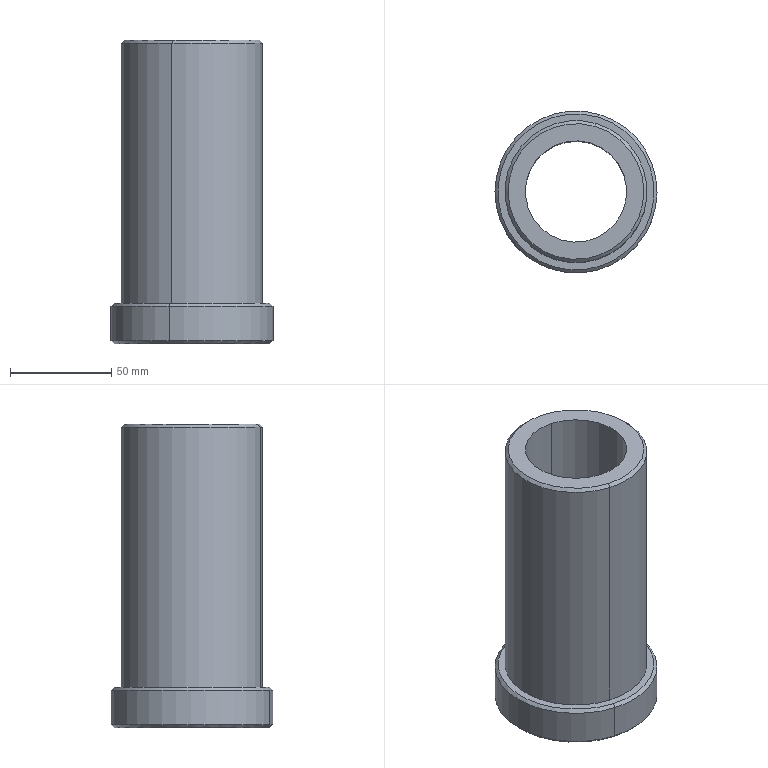Component | SolidWorks | GuideBushing-2 | 1 solid | 15 faces | box 80 x 80 x 150 mm | volume 305503 mm3 | cone 6 | cylinder 6 | plane 3 | commonest cylinder face diameters 50 x2 70 x2 80 x2
build123d program:
from build123d import *

# Parameters (mm, degrees)
CUT_EXTRUDE1_DEPTH      = 161.312
CUT_EXTRUDE1_DEPTH_BACK = 161.312
SKETCH2_R               = 25
CHAMFER1_SIZE           = 1.5


with BuildPart() as part:
    # Sketch1 → Revolve1 (revolve)
    with BuildSketch(Plane.XY, mode=Mode.PRIVATE) as revolve1_sk:
        Polygon((0, 0), (0, 150), (40, 150), (40, 130), (35, 130), (35, 0), align=None)
    revolve(revolve1_sk.sketch.rotate(Axis((0, 0, 0), (0, 1, 0)), 90), axis=Axis((0, 0, 0), (0, 1, 0)))

    # Sketch2 → Cut-Extrude1 (cut, two sides: drawn at the far end of the back side and taken through both)
    with BuildSketch(Plane(origin=(0, 150, 0), x_dir=(1, 0, 0), z_dir=(0, 1, 0)).offset(-CUT_EXTRUDE1_DEPTH_BACK)):
        with Locations(Location((0, 0, 0), (0, 0, 270))):
            Circle(SKETCH2_R)
    extrude(amount=CUT_EXTRUDE1_DEPTH + CUT_EXTRUDE1_DEPTH_BACK, mode=Mode.SUBTRACT)

    # Chamfer1
    chamfer1_edges = [part.edges().sort_by_distance(p)[0] for p in [
        (0, 0, 35),
        (0, 130, 40),
        (0, 150, 40),
    ]]
    chamfer(chamfer1_edges, length=CHAMFER1_SIZE)


solid = part.part

# Placed as in the assembly
solid = solid.moved(Location((-195, 195, -191), (-90, 0, 0)))
STEP:
#1=CARTESIAN_POINT('',(-7.248,9.131,-13.425));
#2=VERTEX_POINT('',#1);
#3=CARTESIAN_POINT('',(-8.106,6.223,-13.425));
#4=VERTEX_POINT('',#3);
#5=CARTESIAN_POINT('',(-7.677,7.677,-13.425));
#6=DIRECTION('',(-0.,0.,-1.));
#7=DIRECTION('',(0.283,0.9591,0.));
#8=AXIS2_PLACEMENT_3D('',#5,#6,#7);
#9=CIRCLE('',#8,1.516);
#10=EDGE_CURVE('',#2,#4,#9,.T.);
#11=ORIENTED_EDGE('',*,*,#10,.F.);
#12=CARTESIAN_POINT('',(-7.232,9.188,-13.366));
#13=VERTEX_POINT('',#12);
#14=CARTESIAN_POINT('',(-7.232,9.188,-13.366));
#15=DIRECTION('',(0.2001,0.6782,0.7071));
#16=VECTOR('',#15,39.37);
#17=LINE('',#14,#16);
#18=EDGE_CURVE('',#2,#13,#17,.T.);
#19=ORIENTED_EDGE('',*,*,#18,.T.);
#20=CARTESIAN_POINT('',(-8.123,6.167,-13.366));
#21=VERTEX_POINT('',#20);
#22=CARTESIAN_POINT('',(-7.677,7.677,-13.366));
#23=DIRECTION('',(0.,-0.,1.));
#24=DIRECTION('',(0.283,0.9591,0.));
#25=AXIS2_PLACEMENT_3D('',#22,#23,#24);
#26=CIRCLE('',#25,1.575);
#27=EDGE_CURVE('',#21,#13,#26,.T.);
#28=ORIENTED_EDGE('',*,*,#27,.F.);
#29=CARTESIAN_POINT('',(-8.123,6.167,-13.366));
#30=DIRECTION('',(-0.2001,-0.6782,0.7071));
#31=VECTOR('',#30,39.37);
#32=LINE('',#29,#31);
#33=EDGE_CURVE('',#4,#21,#32,.T.);
#34=ORIENTED_EDGE('',*,*,#33,.F.);
#35=EDGE_LOOP('',(#11,#19,#28,#34));
#36=FACE_OUTER_BOUND('',#35,.T.);
#37=CARTESIAN_POINT('',(-7.677,7.677,-13.366));
#38=DIRECTION('',(0.,-0.,1.));
#39=DIRECTION('',(-0.283,-0.9591,0.));
#40=AXIS2_PLACEMENT_3D('',#37,#38,#39);
#41=CONICAL_SURFACE('',#40,1.575,0.7854);
#42=ADVANCED_FACE('',(#36),#41,.T.);
#43=CARTESIAN_POINT('',(-8.106,6.223,-12.638));
#44=VERTEX_POINT('',#43);
#45=CARTESIAN_POINT('',(-7.248,9.131,-12.638));
#46=VERTEX_POINT('',#45);
#47=CARTESIAN_POINT('',(-7.677,7.677,-12.638));
#48=DIRECTION('',(0.,-0.,1.));
#49=DIRECTION('',(-0.283,-0.9591,0.));
#50=AXIS2_PLACEMENT_3D('',#47,#48,#49);
#51=CIRCLE('',#50,1.516);
#52=EDGE_CURVE('',#44,#46,#51,.T.);
#53=ORIENTED_EDGE('',*,*,#52,.F.);
#54=CARTESIAN_POINT('',(-8.123,6.167,-12.697));
#55=VERTEX_POINT('',#54);
#56=CARTESIAN_POINT('',(-8.106,6.223,-12.638));
#57=DIRECTION('',(-0.2001,-0.6782,-0.7071));
#58=VECTOR('',#57,39.37);
#59=LINE('',#56,#58);
#60=EDGE_CURVE('',#44,#55,#59,.T.);
#61=ORIENTED_EDGE('',*,*,#60,.T.);
#62=CARTESIAN_POINT('',(-7.232,9.188,-12.697));
#63=VERTEX_POINT('',#62);
#64=CARTESIAN_POINT('',(-7.677,7.677,-12.697));
#65=DIRECTION('',(-0.,0.,-1.));
#66=DIRECTION('',(-0.283,-0.9591,0.));
#67=AXIS2_PLACEMENT_3D('',#64,#65,#66);
#68=CIRCLE('',#67,1.575);
#69=EDGE_CURVE('',#63,#55,#68,.T.);
#70=ORIENTED_EDGE('',*,*,#69,.F.);
#71=CARTESIAN_POINT('',(-7.248,9.131,-12.638));
#72=DIRECTION('',(0.2001,0.6782,-0.7071));
#73=VECTOR('',#72,39.37);
#74=LINE('',#71,#73);
#75=EDGE_CURVE('',#46,#63,#74,.T.);
#76=ORIENTED_EDGE('',*,*,#75,.F.);
#77=EDGE_LOOP('',(#53,#61,#70,#76));
#78=FACE_OUTER_BOUND('',#77,.T.);
#79=CARTESIAN_POINT('',(-7.677,7.677,-12.638));
#80=DIRECTION('',(-0.,0.,-1.));
#81=DIRECTION('',(0.283,0.9591,0.));
#82=AXIS2_PLACEMENT_3D('',#79,#80,#81);
#83=CONICAL_SURFACE('',#82,1.516,0.7854);
#84=ADVANCED_FACE('',(#78),#83,.T.);
#85=CARTESIAN_POINT('',(-8.05,6.412,-7.52));
#86=VERTEX_POINT('',#85);
#87=CARTESIAN_POINT('',(-7.304,8.942,-7.52));
#88=VERTEX_POINT('',#87);
#89=CARTESIAN_POINT('',(-7.677,7.677,-7.52));
#90=DIRECTION('',(0.,-0.,1.));
#91=DIRECTION('',(-0.283,-0.9591,0.));
#92=AXIS2_PLACEMENT_3D('',#89,#90,#91);
#93=CIRCLE('',#92,1.319);
#94=EDGE_CURVE('',#86,#88,#93,.T.);
#95=ORIENTED_EDGE('',*,*,#94,.F.);
#96=CARTESIAN_POINT('',(-8.067,6.356,-7.579));
#97=VERTEX_POINT('',#96);
#98=CARTESIAN_POINT('',(-8.05,6.412,-7.52));
#99=DIRECTION('',(-0.2001,-0.6782,-0.7071));
#100=VECTOR('',#99,39.37);
#101=LINE('',#98,#100);
#102=EDGE_CURVE('',#86,#97,#101,.T.);
#103=ORIENTED_EDGE('',*,*,#102,.T.);
#104=CARTESIAN_POINT('',(-7.287,8.999,-7.579));
#105=VERTEX_POINT('',#104);
#106=CARTESIAN_POINT('',(-7.677,7.677,-7.579));
#107=DIRECTION('',(-0.,0.,-1.));
#108=DIRECTION('',(-0.283,-0.9591,0.));
#109=AXIS2_PLACEMENT_3D('',#106,#107,#108);
#110=CIRCLE('',#109,1.378);
#111=EDGE_CURVE('',#105,#97,#110,.T.);
#112=ORIENTED_EDGE('',*,*,#111,.F.);
#113=CARTESIAN_POINT('',(-7.304,8.942,-7.52));
#114=DIRECTION('',(0.2001,0.6782,-0.7071));
#115=VECTOR('',#114,39.37);
#116=LINE('',#113,#115);
#117=EDGE_CURVE('',#88,#105,#116,.T.);
#118=ORIENTED_EDGE('',*,*,#117,.F.);
#119=EDGE_LOOP('',(#95,#103,#112,#118));
#120=FACE_OUTER_BOUND('',#119,.T.);
#121=CARTESIAN_POINT('',(-7.677,7.677,-7.52));
#122=DIRECTION('',(-0.,0.,-1.));
#123=DIRECTION('',(0.283,0.9591,0.));
#124=AXIS2_PLACEMENT_3D('',#121,#122,#123);
#125=CONICAL_SURFACE('',#124,1.319,0.7854);
#126=ADVANCED_FACE('',(#120),#125,.T.);
#127=CARTESIAN_POINT('',(-7.956,6.733,-7.52));
#128=VERTEX_POINT('',#127);
#129=CARTESIAN_POINT('',(-7.399,8.621,-7.52));
#130=VERTEX_POINT('',#129);
#131=CARTESIAN_POINT('',(-7.677,7.677,-7.52));
#132=DIRECTION('',(-0.,0.,-1.));
#133=DIRECTION('',(0.283,0.9591,0.));
#134=AXIS2_PLACEMENT_3D('',#131,#132,#133);
#135=CIRCLE('',#134,0.9843);
#136=EDGE_CURVE('',#128,#130,#135,.T.);
#137=ORIENTED_EDGE('',*,*,#136,.F.);
#138=CARTESIAN_POINT('',(-7.956,6.733,-13.425));
#139=VERTEX_POINT('',#138);
#140=CARTESIAN_POINT('',(-7.956,6.733,-7.52));
#141=DIRECTION('',(-0.,0.,-1.));
#142=VECTOR('',#141,39.37);
#143=LINE('',#140,#142);
#144=EDGE_CURVE('',#128,#139,#143,.T.);
#145=ORIENTED_EDGE('',*,*,#144,.T.);
#146=CARTESIAN_POINT('',(-7.399,8.621,-13.425));
#147=VERTEX_POINT('',#146);
#148=CARTESIAN_POINT('',(-7.677,7.677,-13.425));
#149=DIRECTION('',(-0.,0.,-1.));
#150=DIRECTION('',(0.283,0.9591,0.));
#151=AXIS2_PLACEMENT_3D('',#148,#149,#150);
#152=CIRCLE('',#151,0.9843);
#153=EDGE_CURVE('',#139,#147,#152,.T.);
#154=ORIENTED_EDGE('',*,*,#153,.T.);
#155=CARTESIAN_POINT('',(-7.399,8.621,-7.52));
#156=DIRECTION('',(-0.,0.,-1.));
#157=VECTOR('',#156,39.37);
#158=LINE('',#155,#157);
#159=EDGE_CURVE('',#130,#147,#158,.T.);
#160=ORIENTED_EDGE('',*,*,#159,.F.);
#161=EDGE_LOOP('',(#137,#145,#154,#160));
#162=FACE_OUTER_BOUND('',#161,.T.);
#163=CARTESIAN_POINT('',(-7.677,7.677,-7.52));
#164=DIRECTION('',(-0.,0.,-1.));
#165=DIRECTION('',(0.283,0.9591,0.));
#166=AXIS2_PLACEMENT_3D('',#163,#164,#165);
#167=CYLINDRICAL_SURFACE('',#166,0.9843);
#168=ADVANCED_FACE('',(#162),#167,.F.);
#169=CARTESIAN_POINT('',(-8.067,6.356,-12.638));
#170=VERTEX_POINT('',#169);
#171=CARTESIAN_POINT('',(-7.287,8.999,-12.638));
#172=VERTEX_POINT('',#171);
#173=CARTESIAN_POINT('',(-7.677,7.677,-12.638));
#174=DIRECTION('',(0.,-0.,1.));
#175=DIRECTION('',(-0.283,-0.9591,0.));
#176=AXIS2_PLACEMENT_3D('',#173,#174,#175);
#177=CIRCLE('',#176,1.378);
#178=EDGE_CURVE('',#170,#172,#177,.T.);
#179=ORIENTED_EDGE('',*,*,#178,.T.);
#180=CARTESIAN_POINT('',(-7.287,8.999,-7.52));
#181=DIRECTION('',(0.,-0.,1.));
#182=VECTOR('',#181,39.37);
#183=LINE('',#180,#182);
#184=EDGE_CURVE('',#172,#105,#183,.T.);
#185=ORIENTED_EDGE('',*,*,#184,.T.);
#186=ORIENTED_EDGE('',*,*,#111,.T.);
#187=CARTESIAN_POINT('',(-8.067,6.356,-7.52));
#188=DIRECTION('',(0.,-0.,1.));
#189=VECTOR('',#188,39.37);
#190=LINE('',#187,#189);
#191=EDGE_CURVE('',#170,#97,#190,.T.);
#192=ORIENTED_EDGE('',*,*,#191,.F.);
#193=EDGE_LOOP('',(#179,#185,#186,#192));
#194=FACE_OUTER_BOUND('',#193,.T.);
#195=CARTESIAN_POINT('',(-7.677,7.677,-7.52));
#196=DIRECTION('',(0.,-0.,1.));
#197=DIRECTION('',(-0.283,-0.9591,0.));
#198=AXIS2_PLACEMENT_3D('',#195,#196,#197);
#199=CYLINDRICAL_SURFACE('',#198,1.378);
#200=ADVANCED_FACE('',(#194),#199,.T.);
#201=ORIENTED_EDGE('',*,*,#27,.T.);
#202=CARTESIAN_POINT('',(-7.232,9.188,-7.52));
#203=DIRECTION('',(0.,-0.,1.));
#204=VECTOR('',#203,39.37);
#205=LINE('',#202,#204);
#206=EDGE_CURVE('',#13,#63,#205,.T.);
#207=ORIENTED_EDGE('',*,*,#206,.T.);
#208=ORIENTED_EDGE('',*,*,#69,.T.);
#209=CARTESIAN_POINT('',(-8.123,6.167,-7.52));
#210=DIRECTION('',(0.,-0.,1.));
#211=VECTOR('',#210,39.37);
#212=LINE('',#209,#211);
#213=EDGE_CURVE('',#21,#55,#212,.T.);
#214=ORIENTED_EDGE('',*,*,#213,.F.);
#215=EDGE_LOOP('',(#201,#207,#208,#214));
#216=FACE_OUTER_BOUND('',#215,.T.);
#217=CARTESIAN_POINT('',(-7.677,7.677,-7.52));
#218=DIRECTION('',(0.,-0.,1.));
#219=DIRECTION('',(-0.283,-0.9591,0.));
#220=AXIS2_PLACEMENT_3D('',#217,#218,#219);
#221=CYLINDRICAL_SURFACE('',#220,1.575);
#222=ADVANCED_FACE('',(#216),#221,.T.);
#223=CARTESIAN_POINT('',(-7.677,7.677,-7.52));
#224=DIRECTION('',(0.,-0.,1.));
#225=DIRECTION('',(-0.283,-0.9591,0.));
#226=AXIS2_PLACEMENT_3D('',#223,#224,#225);
#227=CIRCLE('',#226,1.319);
#228=EDGE_CURVE('',#88,#86,#227,.T.);
#229=ORIENTED_EDGE('',*,*,#228,.T.);
#230=ORIENTED_EDGE('',*,*,#94,.T.);
#231=EDGE_LOOP('',(#229,#230));
#232=FACE_OUTER_BOUND('',#231,.T.);
#233=CARTESIAN_POINT('',(-7.677,7.677,-7.52));
#234=DIRECTION('',(-0.,0.,-1.));
#235=DIRECTION('',(0.283,0.9591,0.));
#236=AXIS2_PLACEMENT_3D('',#233,#234,#235);
#237=CIRCLE('',#236,0.9843);
#238=EDGE_CURVE('',#130,#128,#237,.T.);
#239=ORIENTED_EDGE('',*,*,#238,.T.);
#240=ORIENTED_EDGE('',*,*,#136,.T.);
#241=EDGE_LOOP('',(#239,#240));
#242=FACE_BOUND('',#241,.T.);
#243=CARTESIAN_POINT('',(-6.356,7.287,-7.52));
#244=DIRECTION('',(0.,-0.,1.));
#245=DIRECTION('',(-0.283,-0.9591,0.));
#246=AXIS2_PLACEMENT_3D('',#243,#244,#245);
#247=PLANE('',#246);
#248=ADVANCED_FACE('',(#232,#242),#247,.T.);
#249=CARTESIAN_POINT('',(-7.677,7.677,-13.425));
#250=DIRECTION('',(-0.,0.,-1.));
#251=DIRECTION('',(0.283,0.9591,0.));
#252=AXIS2_PLACEMENT_3D('',#249,#250,#251);
#253=CIRCLE('',#252,1.516);
#254=EDGE_CURVE('',#4,#2,#253,.T.);
#255=ORIENTED_EDGE('',*,*,#254,.T.);
#256=ORIENTED_EDGE('',*,*,#10,.T.);
#257=EDGE_LOOP('',(#255,#256));
#258=FACE_OUTER_BOUND('',#257,.T.);
#259=CARTESIAN_POINT('',(-7.677,7.677,-13.425));
#260=DIRECTION('',(-0.,0.,-1.));
#261=DIRECTION('',(0.283,0.9591,0.));
#262=AXIS2_PLACEMENT_3D('',#259,#260,#261);
#263=CIRCLE('',#262,0.9843);
#264=EDGE_CURVE('',#147,#139,#263,.T.);
#265=ORIENTED_EDGE('',*,*,#264,.F.);
#266=ORIENTED_EDGE('',*,*,#153,.F.);
#267=EDGE_LOOP('',(#265,#266));
#268=FACE_BOUND('',#267,.T.);
#269=CARTESIAN_POINT('',(-7.677,7.677,-13.425));
#270=DIRECTION('',(-0.,0.,-1.));
#271=DIRECTION('',(0.283,0.9591,-0.));
#272=AXIS2_PLACEMENT_3D('',#269,#270,#271);
#273=PLANE('',#272);
#274=ADVANCED_FACE('',(#258,#268),#273,.T.);
#275=ORIENTED_EDGE('',*,*,#206,.F.);
#276=CARTESIAN_POINT('',(-7.677,7.677,-13.366));
#277=DIRECTION('',(0.,-0.,1.));
#278=DIRECTION('',(0.283,0.9591,0.));
#279=AXIS2_PLACEMENT_3D('',#276,#277,#278);
#280=CIRCLE('',#279,1.575);
#281=EDGE_CURVE('',#13,#21,#280,.T.);
#282=ORIENTED_EDGE('',*,*,#281,.T.);
#283=ORIENTED_EDGE('',*,*,#213,.T.);
#284=CARTESIAN_POINT('',(-7.677,7.677,-12.697));
#285=DIRECTION('',(-0.,0.,-1.));
#286=DIRECTION('',(-0.283,-0.9591,0.));
#287=AXIS2_PLACEMENT_3D('',#284,#285,#286);
#288=CIRCLE('',#287,1.575);
#289=EDGE_CURVE('',#55,#63,#288,.T.);
#290=ORIENTED_EDGE('',*,*,#289,.T.);
#291=EDGE_LOOP('',(#275,#282,#283,#290));
#292=FACE_OUTER_BOUND('',#291,.T.);
#293=CARTESIAN_POINT('',(-7.677,7.677,-7.52));
#294=DIRECTION('',(0.,-0.,1.));
#295=DIRECTION('',(-0.283,-0.9591,0.));
#296=AXIS2_PLACEMENT_3D('',#293,#294,#295);
#297=CYLINDRICAL_SURFACE('',#296,1.575);
#298=ADVANCED_FACE('',(#292),#297,.T.);
#299=CARTESIAN_POINT('',(-7.677,7.677,-12.638));
#300=DIRECTION('',(0.,-0.,1.));
#301=DIRECTION('',(-0.283,-0.9591,0.));
#302=AXIS2_PLACEMENT_3D('',#299,#300,#301);
#303=CIRCLE('',#302,1.516);
#304=EDGE_CURVE('',#46,#44,#303,.T.);
#305=ORIENTED_EDGE('',*,*,#304,.T.);
#306=ORIENTED_EDGE('',*,*,#52,.T.);
#307=EDGE_LOOP('',(#305,#306));
#308=FACE_OUTER_BOUND('',#307,.T.);
#309=ORIENTED_EDGE('',*,*,#178,.F.);
#310=CARTESIAN_POINT('',(-7.677,7.677,-12.638));
#311=DIRECTION('',(0.,-0.,1.));
#312=DIRECTION('',(-0.283,-0.9591,0.));
#313=AXIS2_PLACEMENT_3D('',#310,#311,#312);
#314=CIRCLE('',#313,1.378);
#315=EDGE_CURVE('',#172,#170,#314,.T.);
#316=ORIENTED_EDGE('',*,*,#315,.F.);
#317=EDGE_LOOP('',(#309,#316));
#318=FACE_BOUND('',#317,.T.);
#319=CARTESIAN_POINT('',(-6.167,7.232,-12.638));
#320=DIRECTION('',(0.,-0.,1.));
#321=DIRECTION('',(-0.283,-0.9591,0.));
#322=AXIS2_PLACEMENT_3D('',#319,#320,#321);
#323=PLANE('',#322);
#324=ADVANCED_FACE('',(#308,#318),#323,.T.);
#325=ORIENTED_EDGE('',*,*,#184,.F.);
#326=ORIENTED_EDGE('',*,*,#315,.T.);
#327=ORIENTED_EDGE('',*,*,#191,.T.);
#328=CARTESIAN_POINT('',(-7.677,7.677,-7.579));
#329=DIRECTION('',(-0.,0.,-1.));
#330=DIRECTION('',(-0.283,-0.9591,0.));
#331=AXIS2_PLACEMENT_3D('',#328,#329,#330);
#332=CIRCLE('',#331,1.378);
#333=EDGE_CURVE('',#97,#105,#332,.T.);
#334=ORIENTED_EDGE('',*,*,#333,.T.);
#335=EDGE_LOOP('',(#325,#326,#327,#334));
#336=FACE_OUTER_BOUND('',#335,.T.);
#337=CARTESIAN_POINT('',(-7.677,7.677,-7.52));
#338=DIRECTION('',(0.,-0.,1.));
#339=DIRECTION('',(-0.283,-0.9591,0.));
#340=AXIS2_PLACEMENT_3D('',#337,#338,#339);
#341=CYLINDRICAL_SURFACE('',#340,1.378);
#342=ADVANCED_FACE('',(#336),#341,.T.);
#343=ORIENTED_EDGE('',*,*,#144,.F.);
#344=ORIENTED_EDGE('',*,*,#238,.F.);
#345=ORIENTED_EDGE('',*,*,#159,.T.);
#346=ORIENTED_EDGE('',*,*,#264,.T.);
#347=EDGE_LOOP('',(#343,#344,#345,#346));
#348=FACE_OUTER_BOUND('',#347,.T.);
#349=CARTESIAN_POINT('',(-7.677,7.677,-7.52));
#350=DIRECTION('',(-0.,0.,-1.));
#351=DIRECTION('',(0.283,0.9591,0.));
#352=AXIS2_PLACEMENT_3D('',#349,#350,#351);
#353=CYLINDRICAL_SURFACE('',#352,0.9843);
#354=ADVANCED_FACE('',(#348),#353,.F.);
#355=ORIENTED_EDGE('',*,*,#102,.F.);
#356=ORIENTED_EDGE('',*,*,#228,.F.);
#357=ORIENTED_EDGE('',*,*,#117,.T.);
#358=ORIENTED_EDGE('',*,*,#333,.F.);
#359=EDGE_LOOP('',(#355,#356,#357,#358));
#360=FACE_OUTER_BOUND('',#359,.T.);
#361=CARTESIAN_POINT('',(-7.677,7.677,-7.52));
#362=DIRECTION('',(-0.,0.,-1.));
#363=DIRECTION('',(0.283,0.9591,0.));
#364=AXIS2_PLACEMENT_3D('',#361,#362,#363);
#365=CONICAL_SURFACE('',#364,1.319,0.7854);
#366=ADVANCED_FACE('',(#360),#365,.T.);
#367=ORIENTED_EDGE('',*,*,#60,.F.);
#368=ORIENTED_EDGE('',*,*,#304,.F.);
#369=ORIENTED_EDGE('',*,*,#75,.T.);
#370=ORIENTED_EDGE('',*,*,#289,.F.);
#371=EDGE_LOOP('',(#367,#368,#369,#370));
#372=FACE_OUTER_BOUND('',#371,.T.);
#373=CARTESIAN_POINT('',(-7.677,7.677,-12.638));
#374=DIRECTION('',(-0.,0.,-1.));
#375=DIRECTION('',(0.283,0.9591,0.));
#376=AXIS2_PLACEMENT_3D('',#373,#374,#375);
#377=CONICAL_SURFACE('',#376,1.516,0.7854);
#378=ADVANCED_FACE('',(#372),#377,.T.);
#379=ORIENTED_EDGE('',*,*,#18,.F.);
#380=ORIENTED_EDGE('',*,*,#254,.F.);
#381=ORIENTED_EDGE('',*,*,#33,.T.);
#382=ORIENTED_EDGE('',*,*,#281,.F.);
#383=EDGE_LOOP('',(#379,#380,#381,#382));
#384=FACE_OUTER_BOUND('',#383,.T.);
#385=CARTESIAN_POINT('',(-7.677,7.677,-13.366));
#386=DIRECTION('',(0.,-0.,1.));
#387=DIRECTION('',(-0.283,-0.9591,0.));
#388=AXIS2_PLACEMENT_3D('',#385,#386,#387);
#389=CONICAL_SURFACE('',#388,1.575,0.7854);
#390=ADVANCED_FACE('',(#384),#389,.T.);
#391=CLOSED_SHELL('',(#42,#84,#126,#168,#200,#222,#248,#274,#298,#324,#342,#354,#366,#378,#390));
#392=MANIFOLD_SOLID_BREP('',#391);
#393=CARTESIAN_POINT('',(0.,0.,0.));
#394=DIRECTION('',(0.,0.,1.));
#395=DIRECTION('',(1.,0.,0.));
#396=AXIS2_PLACEMENT_3D('',#393,#394,#395);
#397=(LENGTH_UNIT()NAMED_UNIT(*)SI_UNIT($,.METRE.));
#398=LENGTH_MEASURE_WITH_UNIT(LENGTH_MEASURE(0.0254),#397);
#399=DIMENSIONAL_EXPONENTS(1.,0.,0.,0.,0.,0.,0.);
#400=(CONVERSION_BASED_UNIT('',#398)LENGTH_UNIT()NAMED_UNIT(#399));
#401=UNCERTAINTY_MEASURE_WITH_UNIT(LENGTH_MEASURE(0.00001),#400,'','');
#402=(NAMED_UNIT(*)PLANE_ANGLE_UNIT()SI_UNIT($,.RADIAN.));
#403=(NAMED_UNIT(*)SI_UNIT($,.STERADIAN.)SOLID_ANGLE_UNIT());
#404=(GEOMETRIC_REPRESENTATION_CONTEXT(3)GLOBAL_UNCERTAINTY_ASSIGNED_CONTEXT((#401))GLOBAL_UNIT_ASSIGNED_CONTEXT((#400,#402,#403))REPRESENTATION_CONTEXT('',''));
#405=ADVANCED_BREP_SHAPE_REPRESENTATION('',(#392,#396),#404);
#406=COLOUR_RGB('',0.7922,0.8196,0.9333);
#407=FILL_AREA_STYLE_COLOUR('',#406);
#408=FILL_AREA_STYLE('',(#407));
#409=SURFACE_STYLE_FILL_AREA(#408);
#410=SURFACE_SIDE_STYLE('',(#409));
#411=SURFACE_STYLE_USAGE(.BOTH.,#410);
#412=PRESENTATION_STYLE_ASSIGNMENT((#411));
#413=STYLED_ITEM('',(#412),#392);
#414=PRESENTATION_LAYER_ASSIGNMENT('','',(#413));
#415=(LENGTH_UNIT()NAMED_UNIT(*)SI_UNIT($,.METRE.));
#416=LENGTH_MEASURE_WITH_UNIT(LENGTH_MEASURE(0.0254),#415);
#417=DIMENSIONAL_EXPONENTS(1.,0.,0.,0.,0.,0.,0.);
#418=(CONVERSION_BASED_UNIT('',#416)LENGTH_UNIT()NAMED_UNIT(#417));
#419=UNCERTAINTY_MEASURE_WITH_UNIT(LENGTH_MEASURE(0.00001),#418,'','');
#420=(NAMED_UNIT(*)PLANE_ANGLE_UNIT()SI_UNIT($,.RADIAN.));
#421=(NAMED_UNIT(*)SI_UNIT($,.STERADIAN.)SOLID_ANGLE_UNIT());
#422=(GEOMETRIC_REPRESENTATION_CONTEXT(3)GLOBAL_UNCERTAINTY_ASSIGNED_CONTEXT((#419))GLOBAL_UNIT_ASSIGNED_CONTEXT((#418,#420,#421))REPRESENTATION_CONTEXT('',''));
#423=MECHANICAL_DESIGN_GEOMETRIC_PRESENTATION_REPRESENTATION('',(#413),#422);